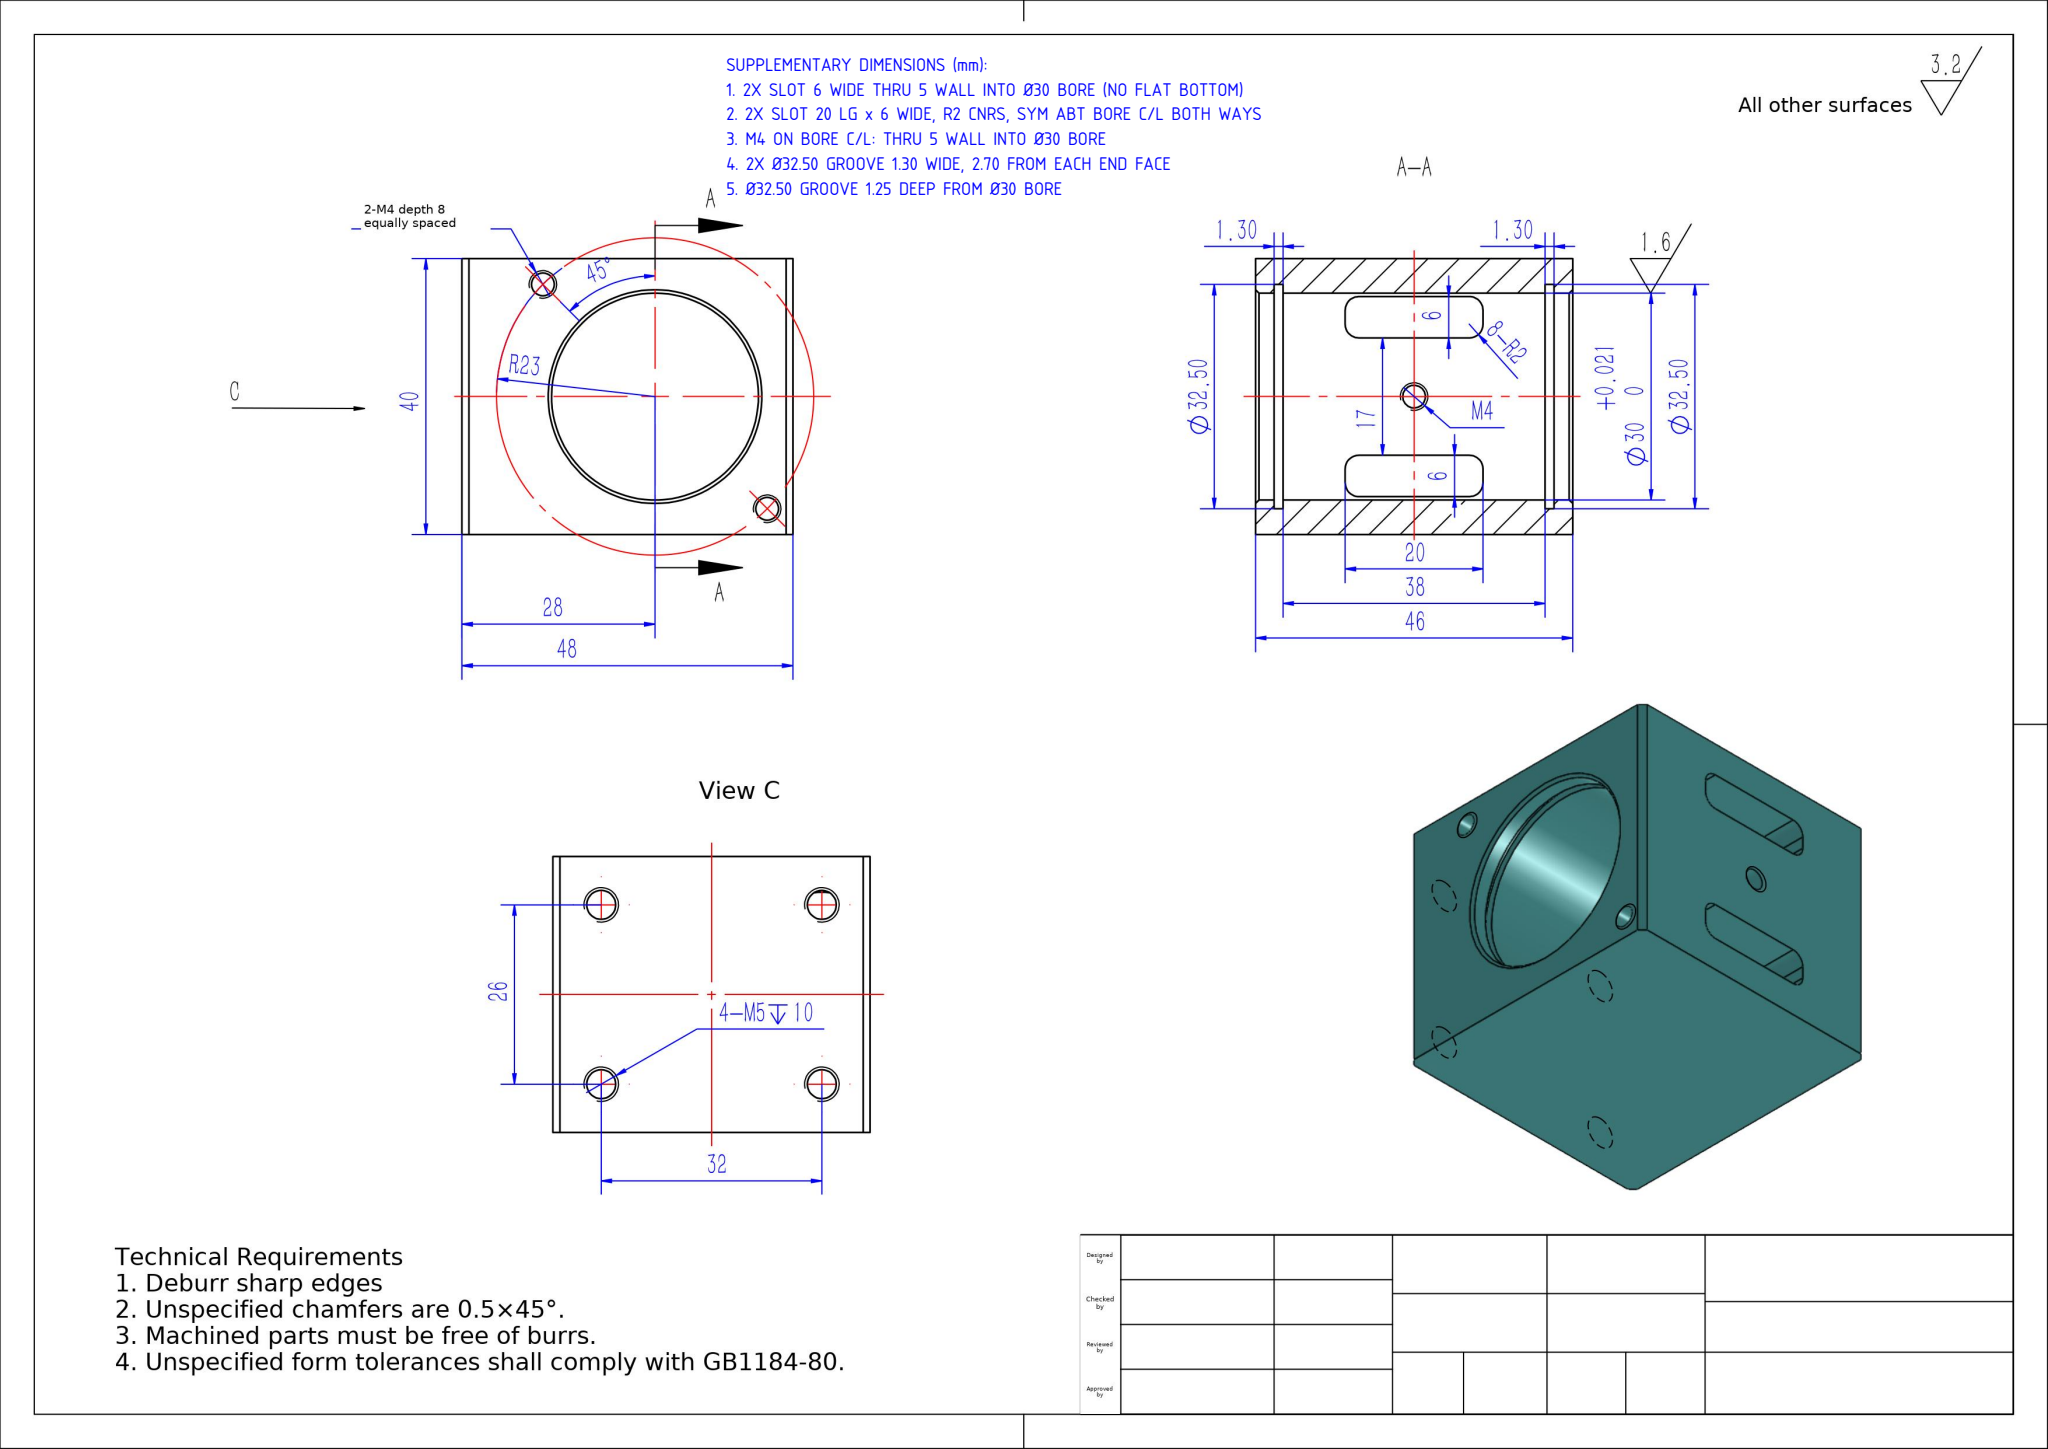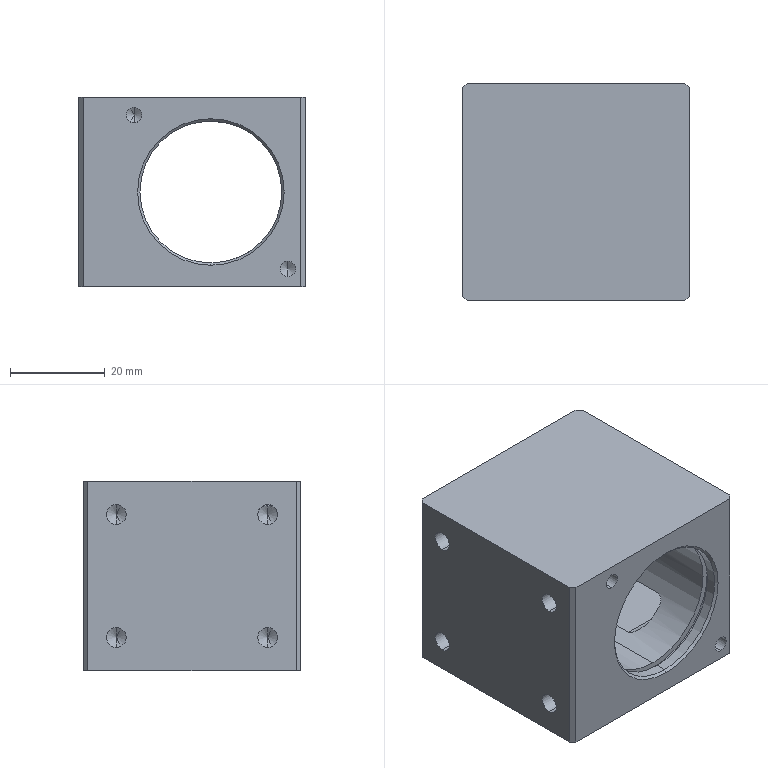Part | SolidWorks | mm | 1 solid | 70 faces | box 48 x 46 x 40 mm | volume 51934 mm3 | cylinder 32 | plane 22 | cone 16 | commonest cylinder face diameters 4.2 x8 4 x8 3.3 x6 30 x6 32.5 x4
build123d program:
from build123d import *

# Parameters (mm, degrees)
SKETCH1_W               = 48
SKETCH1_H               = 40
SKETCH1_R               = 15
BOSS_EXTRUDE1_DEPTH     = 23
SKETCH2_W               = 1.25
SKETCH2_H               = 1.3
CUT_EXTRUDE1_REACH      = 58.859
CUT_EXTRUDE1_END_RADIUS = 15
SKETCH3_W               = 6
SKETCH3_H               = 20
FILLET1_R               = 2
M5_TAPPED_HOLE1_D       = 4.2
M5_TAPPED_HOLE1_DEPTH   = 12.4
M5_TAPPED_HOLE1_TIP     = 1.262
CHAMFER1_SIZE           = 1
CHAMFER2_SIZE           = 0.5
CIRPATTERN1_COUNT       = 2
M4_TAPPED_HOLE2_REACH   = 58.859
M4_TAPPED_HOLE2_BORE_R  = 1.65


with BuildPart() as part:
    # Sketch1 → Boss-Extrude1 (new, symmetric)
    with BuildSketch(Plane(origin=(0, 0, 0), x_dir=(1, 0, 0), z_dir=(0, 1, 0))):
        with Locations((24, 0)):
            Rectangle(SKETCH1_W, SKETCH1_H)
        with Locations(Location((28, 0, 0), (0, 0, 270))):
            Circle(SKETCH1_R, mode=Mode.SUBTRACT)
    extrude(amount=BOSS_EXTRUDE1_DEPTH, both=True)

    # Sketch2 → Cut-Revolve1 (revolve, cut)
    with BuildSketch(Plane.XY):
        with Locations((12.375, -19.65)):
            Rectangle(SKETCH2_W, SKETCH2_H)
        with Locations((12.375, 19.65)):
            Rectangle(SKETCH2_W, SKETCH2_H)
    revolve(axis=Axis((28, 15.897, 0), (0, -1, 0)), mode=Mode.SUBTRACT)

    # Cut-Extrude1: up to this cylinder (the profile starts outside it)
    cut_extrude1_end = Plane(origin=(28, 0, 0), z_dir=(0, -1, 0)) * Cylinder(CUT_EXTRUDE1_END_RADIUS, 148.718, mode=Mode.PRIVATE)
    # Sketch3 → Cut-Extrude1 (cut, up to the surface)
    with BuildSketch(Plane(origin=(48, 0, 0), x_dir=(0, 0, -1), z_dir=(1, 0, 0)), mode=Mode.PRIVATE) as cut_extrude1_sk1:
        with Locations((-11.5, 0)):
            Rectangle(SKETCH3_W, SKETCH3_H)
    cut_extrude1_tool1 = extrude(cut_extrude1_sk1.sketch, amount=-CUT_EXTRUDE1_REACH, mode=Mode.PRIVATE) - cut_extrude1_end
    add(cut_extrude1_tool1.solids().sort_by_distance((48, 0, 11.5))[0], mode=Mode.SUBTRACT)
    # Sketch3 → Cut-Extrude1 (cut, up to the surface)
    with BuildSketch(Plane(origin=(48, 0, 0), x_dir=(0, 0, -1), z_dir=(1, 0, 0)), mode=Mode.PRIVATE) as cut_extrude1_sk2:
        with Locations((11.5, 0)):
            Rectangle(SKETCH3_W, SKETCH3_H)
    cut_extrude1_tool2 = extrude(cut_extrude1_sk2.sketch, amount=-CUT_EXTRUDE1_REACH, mode=Mode.PRIVATE) - cut_extrude1_end
    add(cut_extrude1_tool2.solids().sort_by_distance((48, 0, -11.5))[0], mode=Mode.SUBTRACT)

    # Fillet1
    fillet1_edges = [part.edges().sort_by_distance(p)[0] for p in [
        (44.18, -10, 8.5),
        (44.18, 10, 8.5),
        (39.92, 10, 14.5),
        (39.92, -10, 14.5),
        (44.18, 10, -8.5),
        (44.18, -10, -8.5),
        (39.92, -10, -14.5),
        (39.92, 10, -14.5),
    ]]
    fillet(fillet1_edges, radius=FILLET1_R)

    # M5 Tapped Hole1
    with Locations(Plane.ZY):
        with Locations((-13, 16), (-13, -16), (13, -16), (13, 16)):
            Hole(M5_TAPPED_HOLE1_D / 2, depth=M5_TAPPED_HOLE1_DEPTH)
            with Locations((0, 0, -(M5_TAPPED_HOLE1_DEPTH + M5_TAPPED_HOLE1_TIP / 2))):  # 118° drill point
                Cone(0, M5_TAPPED_HOLE1_D / 2, M5_TAPPED_HOLE1_TIP, mode=Mode.SUBTRACT)

    # Chamfer1
    chamfer1_edges = [part.edges().sort_by_distance(p)[0] for p in [
        (48, 23, 0),
        (0, 23, 0),
        (48, -23, 0),
        (0, -23, 0),
    ]]
    chamfer(chamfer1_edges, length=CHAMFER1_SIZE)

    # Chamfer2
    chamfer2_edges = [part.edges().sort_by_distance(p)[0] for p in [
        (28, -23, -15),
        (28, 23, -15),
    ]]
    chamfer(chamfer2_edges, length=CHAMFER2_SIZE)

    # Sketch9 → M4 Tapped Hole1 (revolve, cut)
    with BuildSketch(Plane(origin=(44.263, -23, -16.263), x_dir=(0, 0, -1), z_dir=(1, 0, 0))):
        Polygon((0, 0), (0, 11.091), (1.65, 10.1), (1.65, 0), align=None)
    m4_tapped_hole1 = revolve(axis=Axis((44.263, -29.35, -16.263), (0, 1, 0)), mode=Mode.SUBTRACT)

    # CirPattern1: M4 Tapped Hole1 ×2 about axis
    cirpattern1_axis = Axis((28, 0, 0), (0, 1, 0))
    for i in range(1, CIRPATTERN1_COUNT):
        add(m4_tapped_hole1.rotate(cirpattern1_axis, i * 360 / CIRPATTERN1_COUNT), mode=Mode.SUBTRACT)

    # M4 Tapped Hole2 bore → M4 Tapped Hole2 (cut, up to next)
    with BuildSketch(Plane(origin=(48, 0, 0), x_dir=(0, 0, -1), z_dir=(1, 0, 0)), mode=Mode.PRIVATE) as m4_tapped_hole2_sk1:
        Circle(M4_TAPPED_HOLE2_BORE_R)
    m4_tapped_hole2_tool1 = extrude(m4_tapped_hole2_sk1.sketch, amount=-M4_TAPPED_HOLE2_REACH, mode=Mode.PRIVATE) & part.part
    add(m4_tapped_hole2_tool1.solids().sort_by_distance((48, 0, 0))[0], mode=Mode.SUBTRACT)


solid = part.part